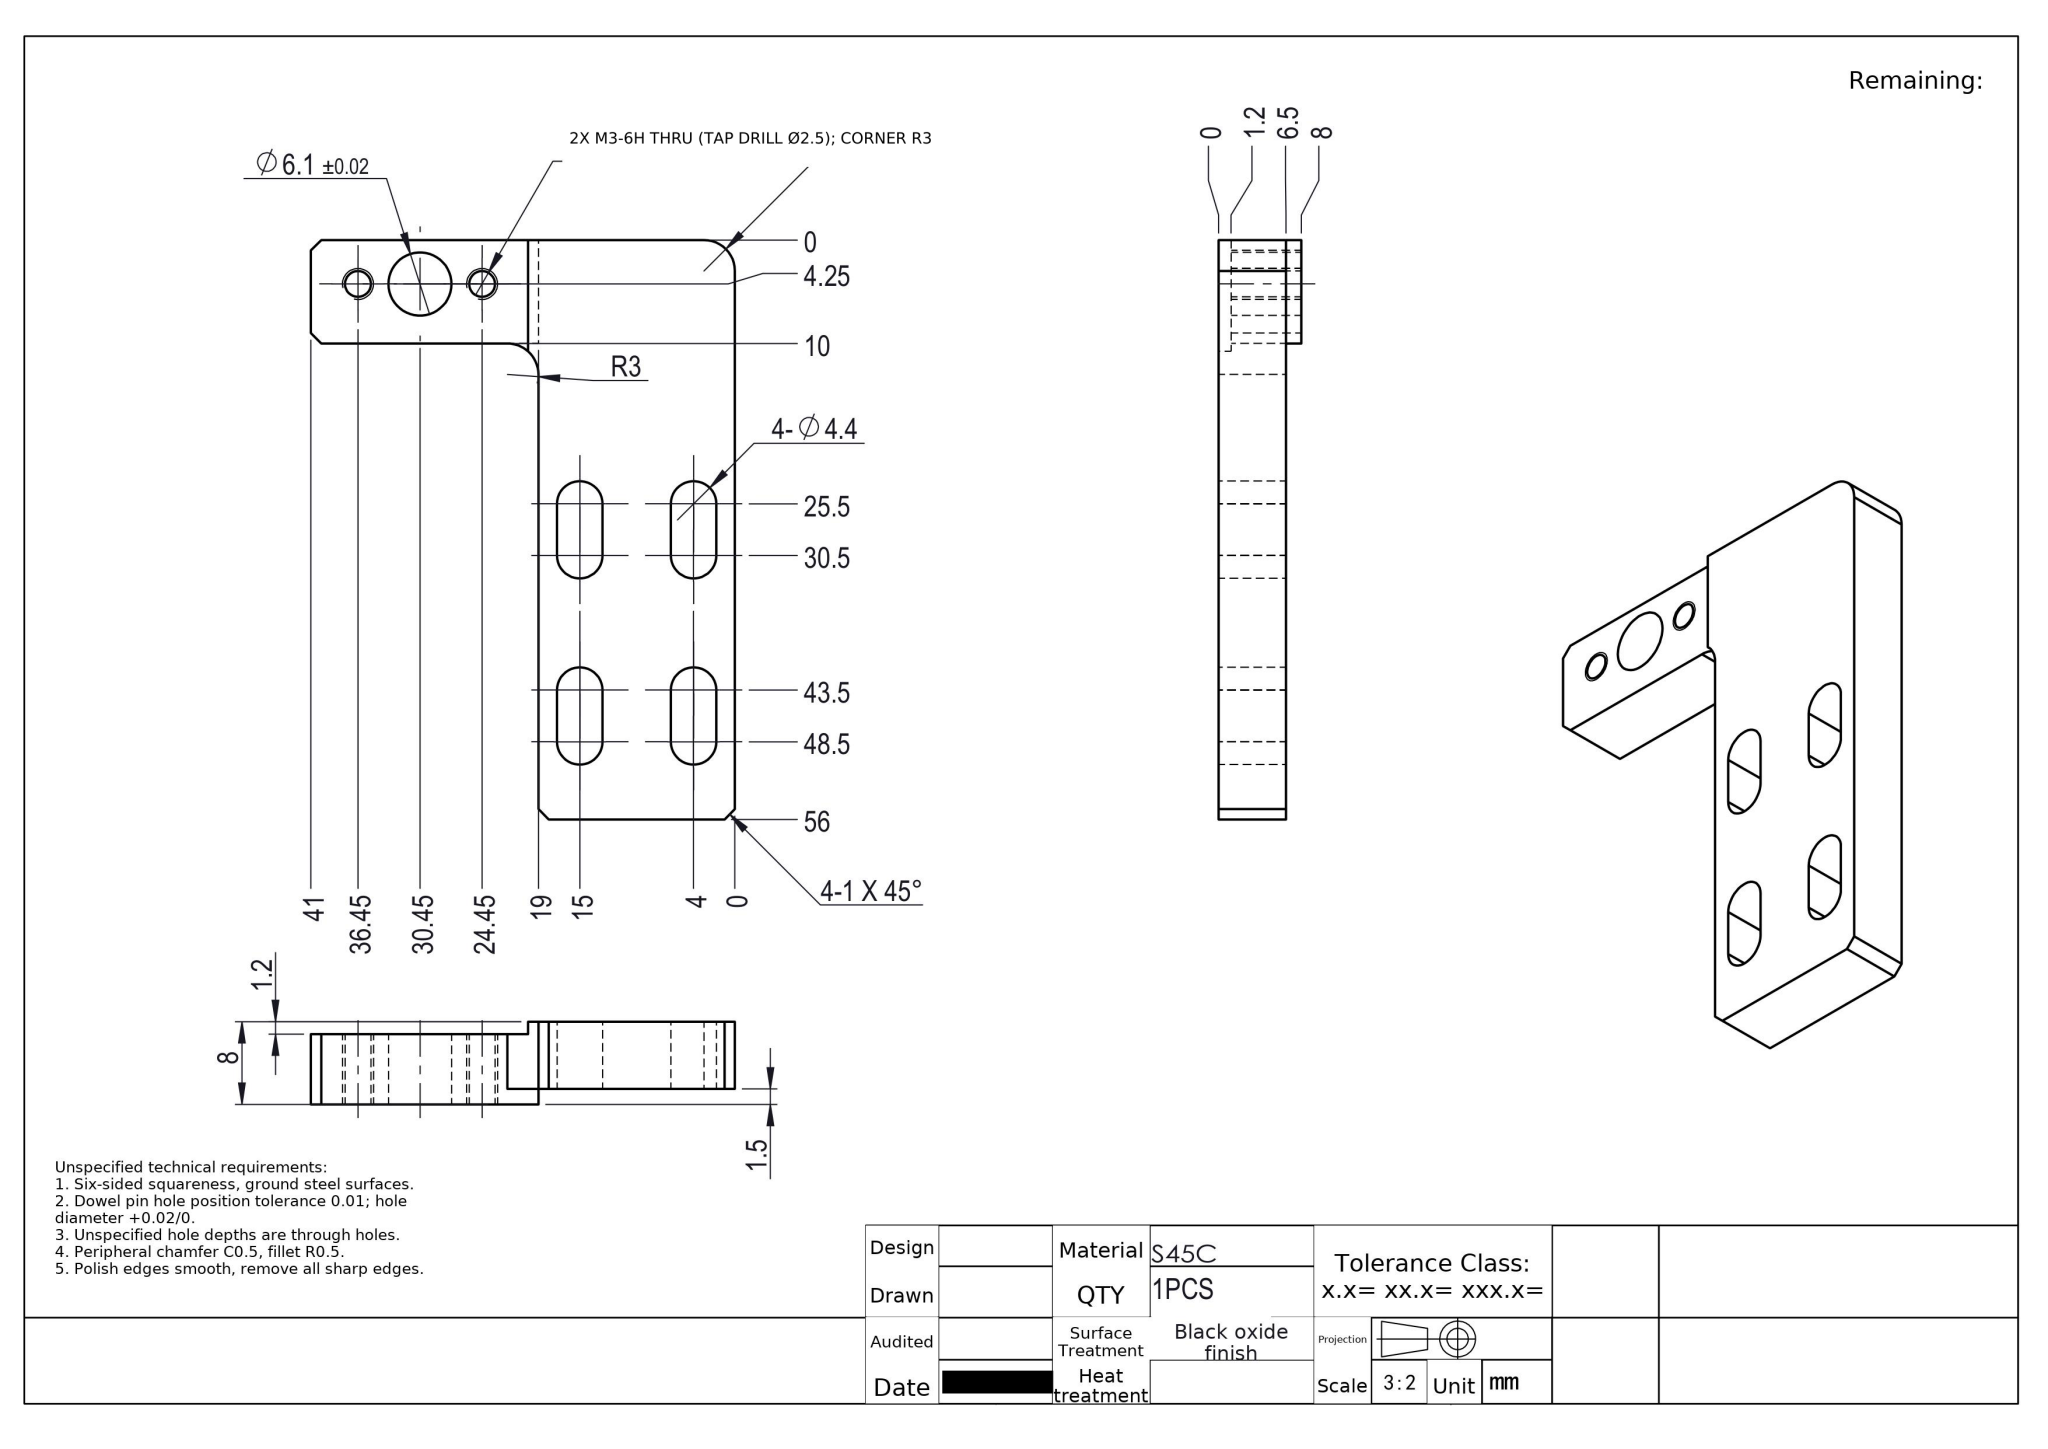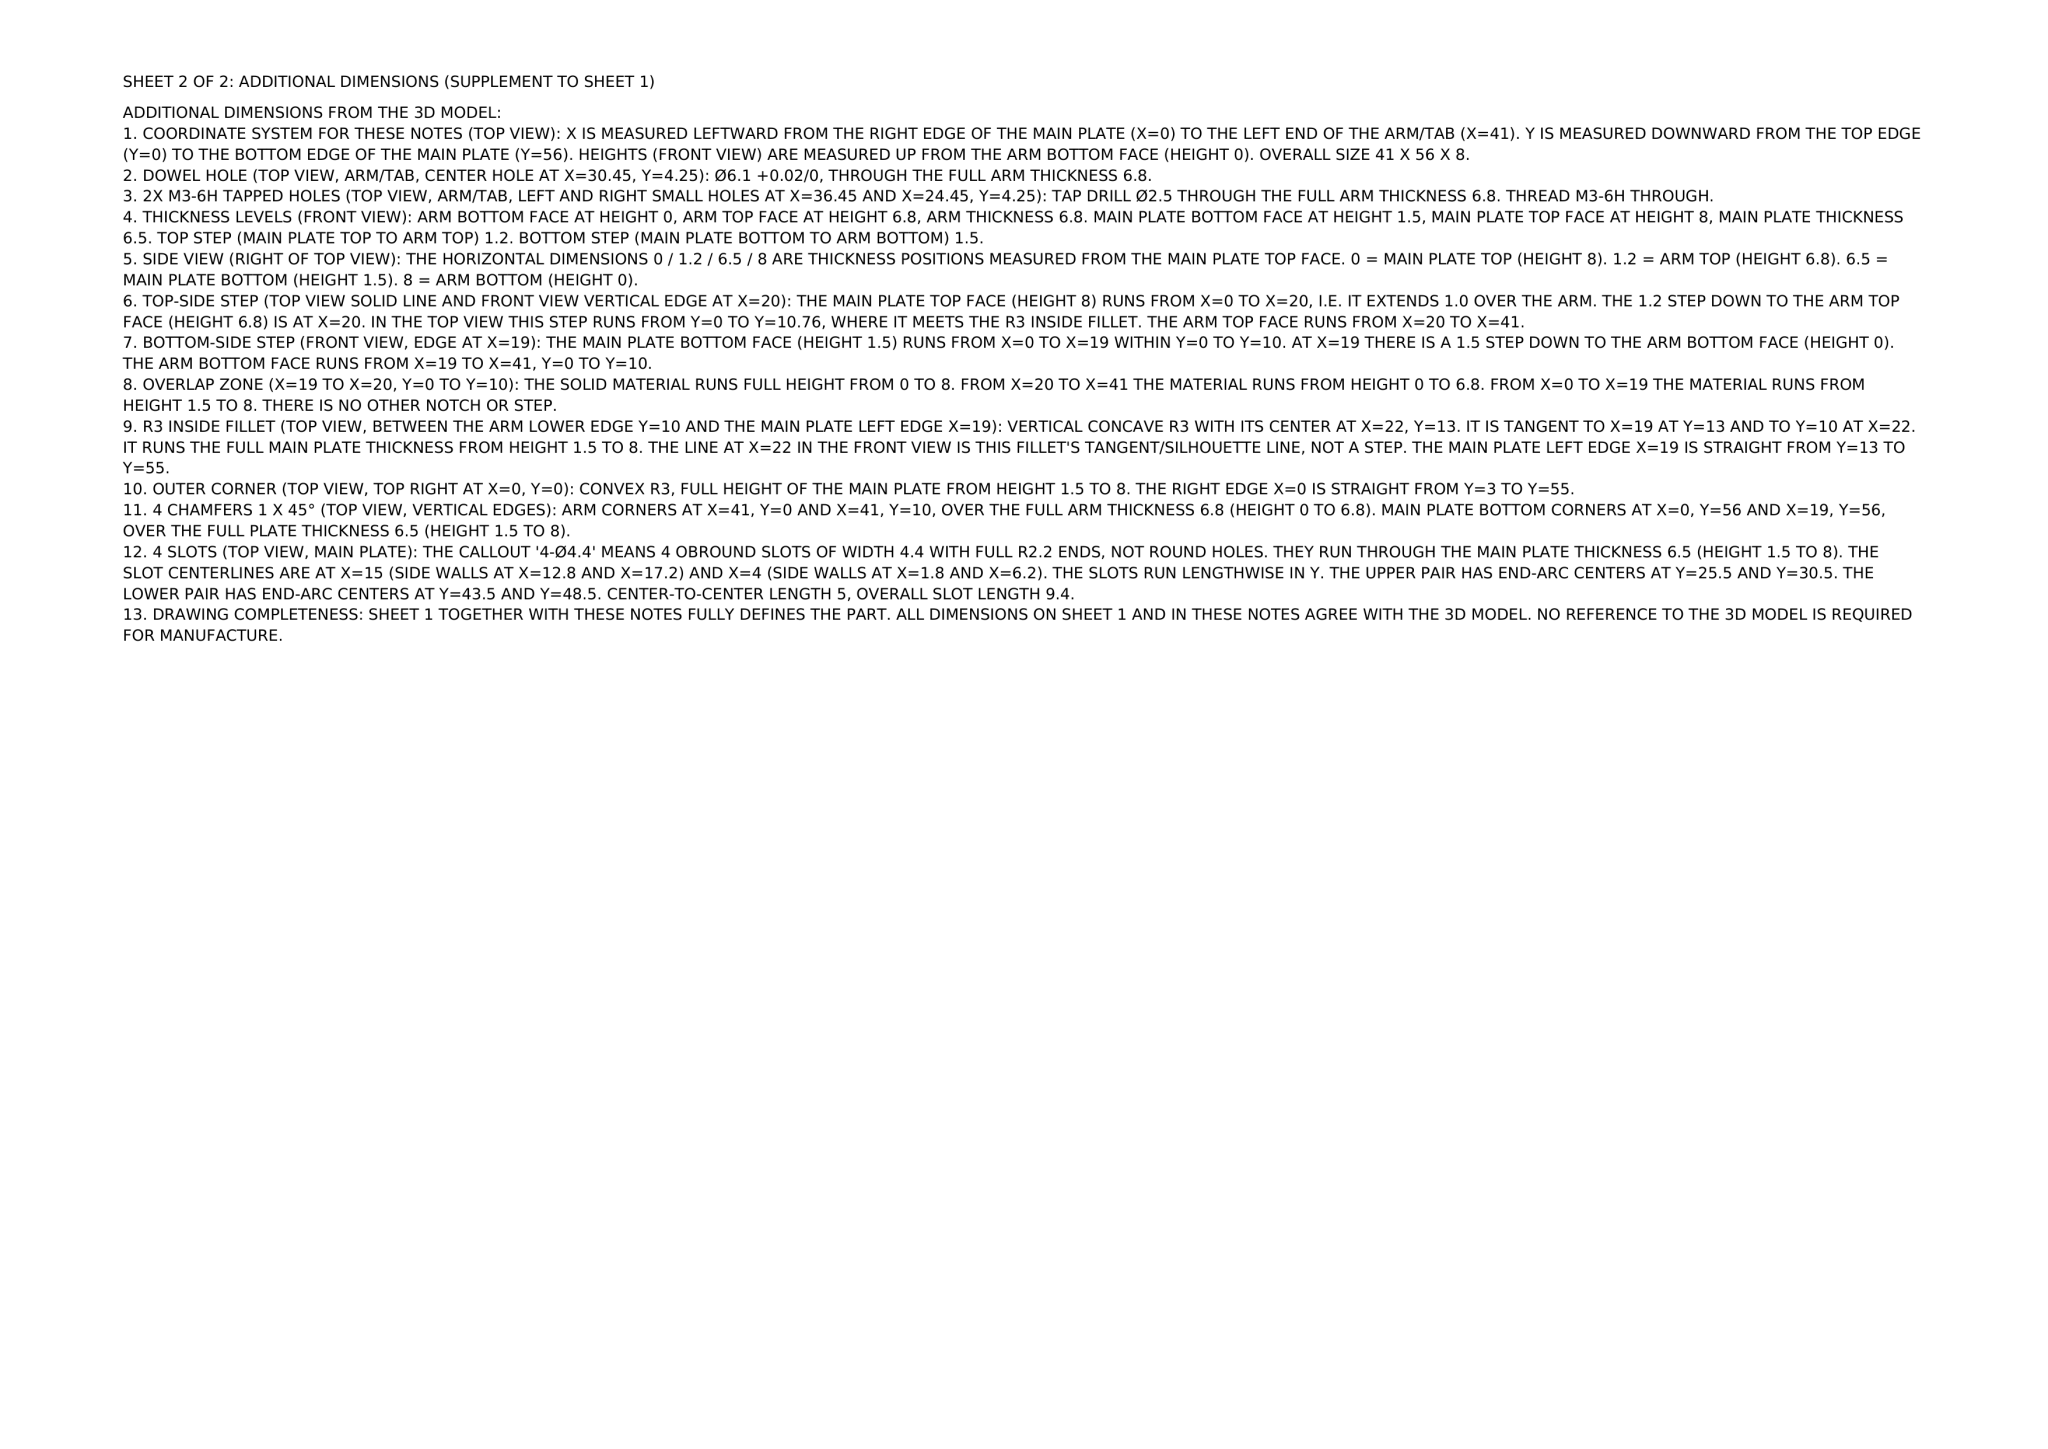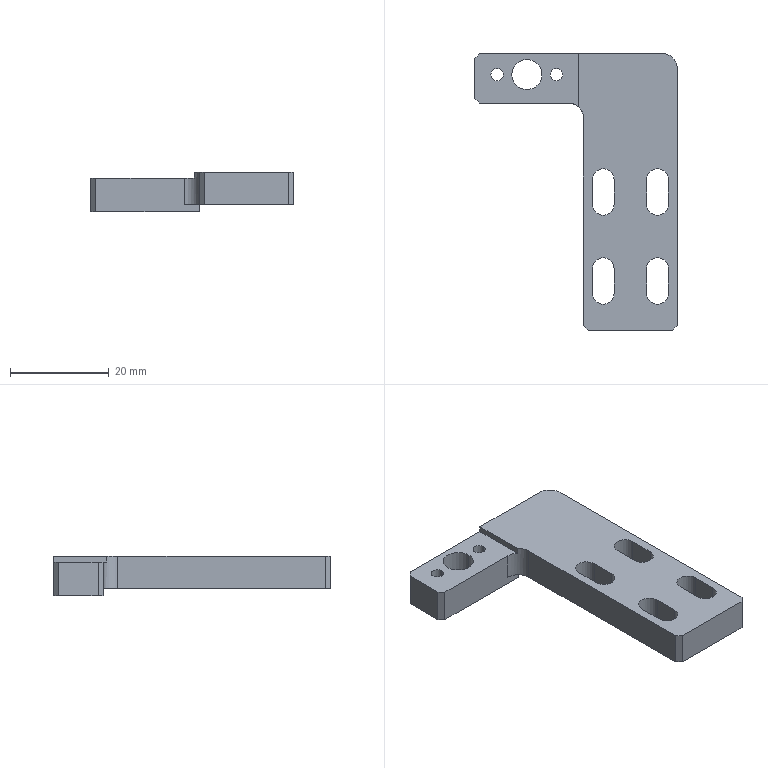Part | NX | mm | 1 solid | 40 faces | box 41 x 56 x 8 mm | volume 7177 mm3 | plane 24 | cylinder 16 | commonest cylinder face diameters 4.4 x8 2.5 x4 6.1 x2 6 x2